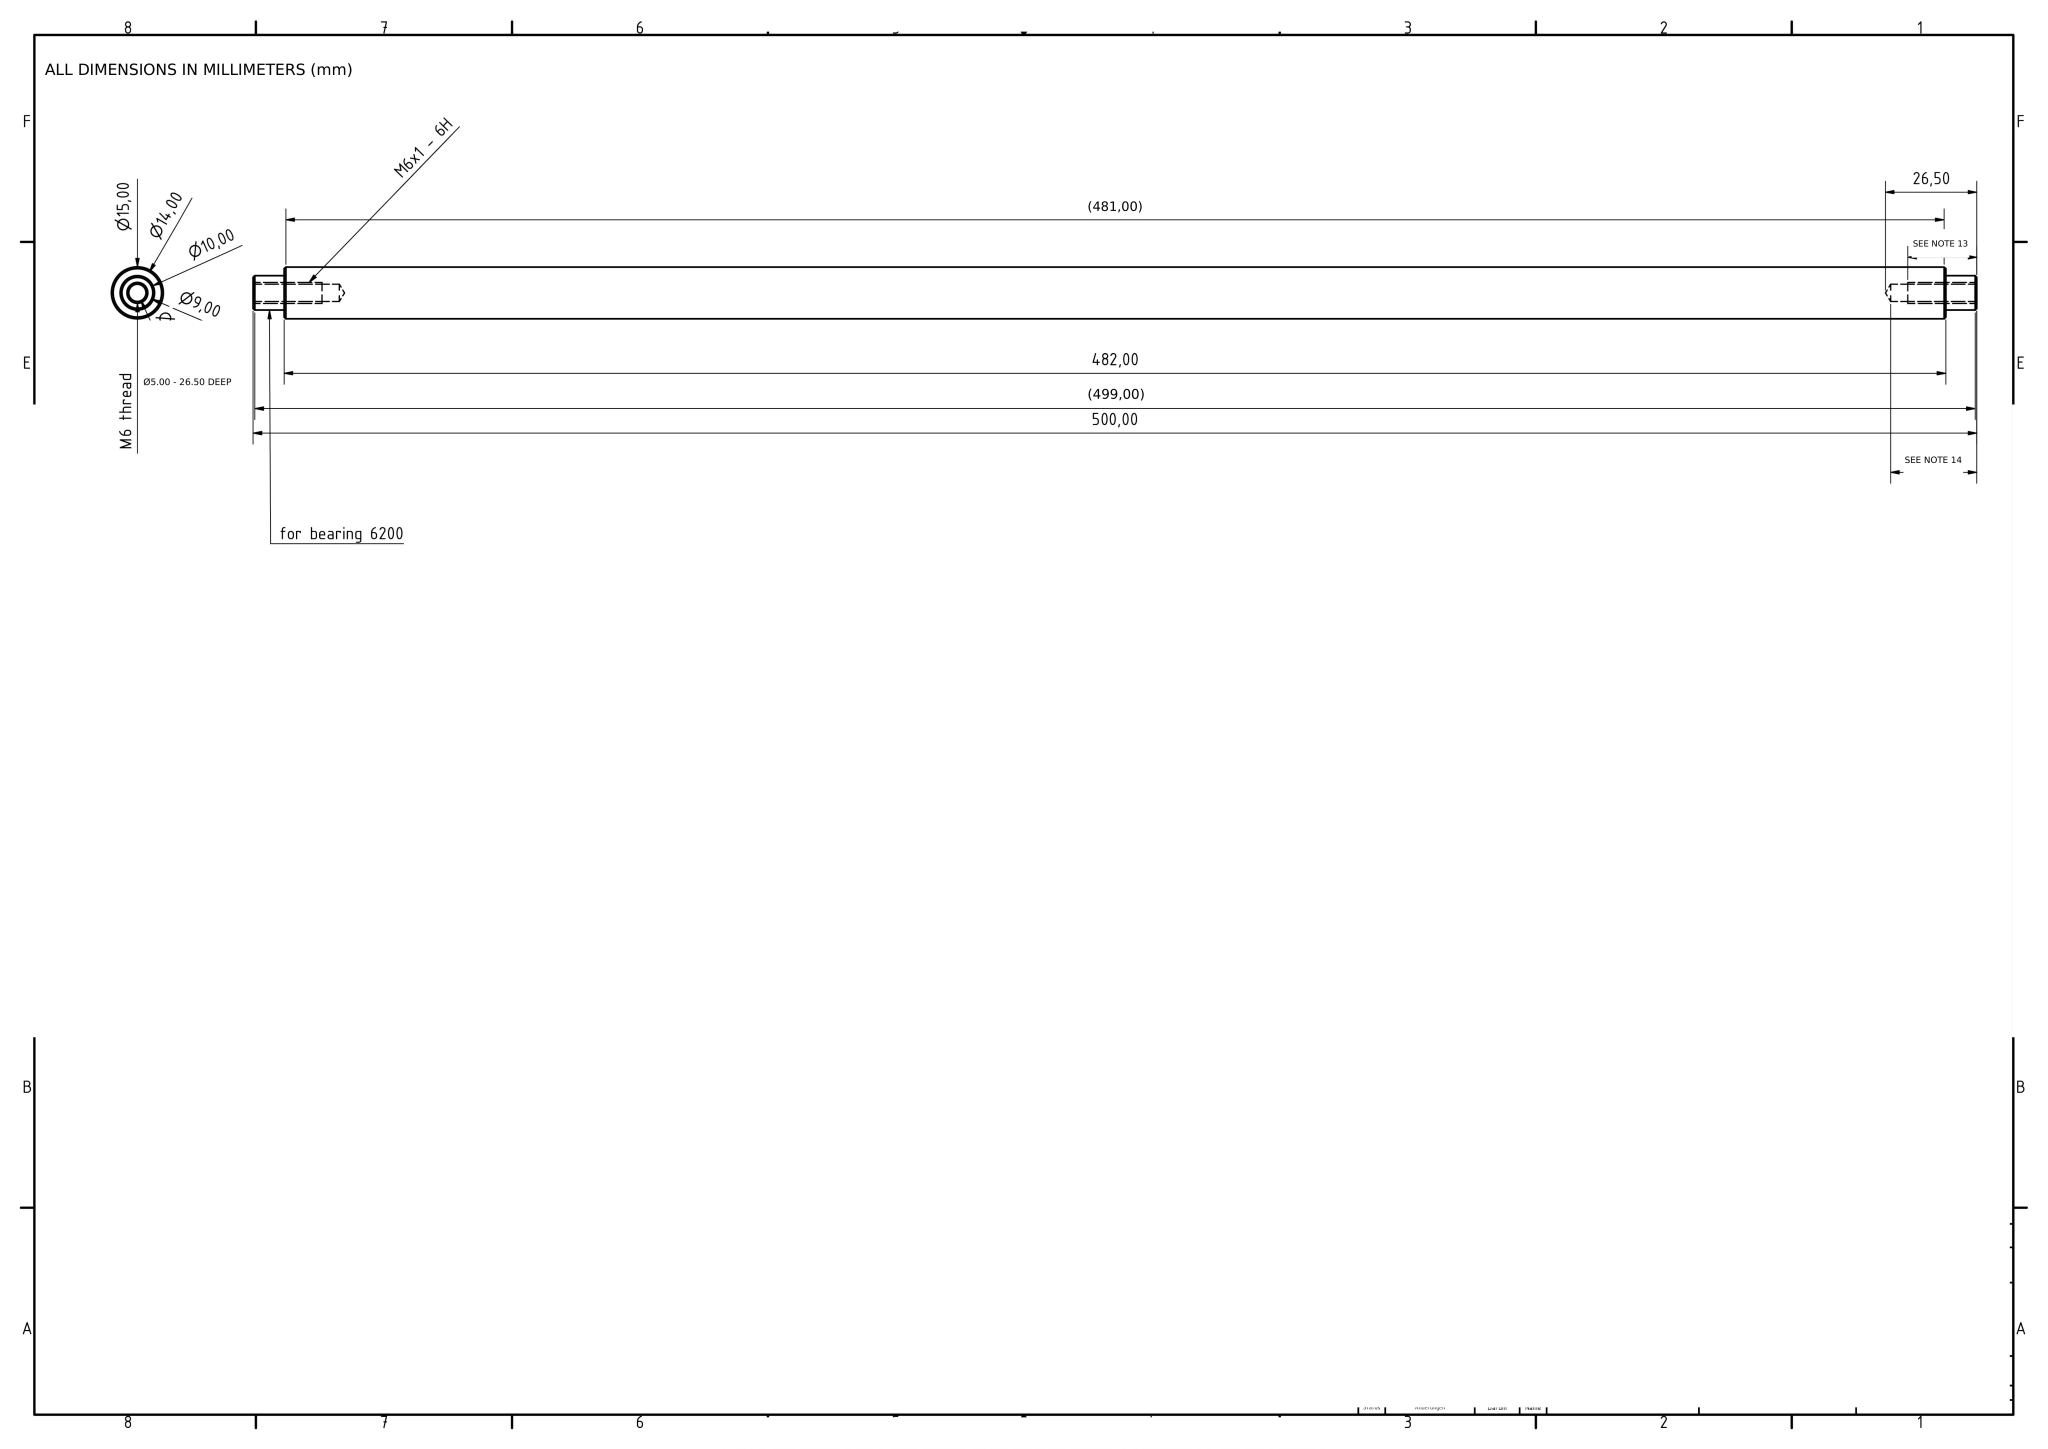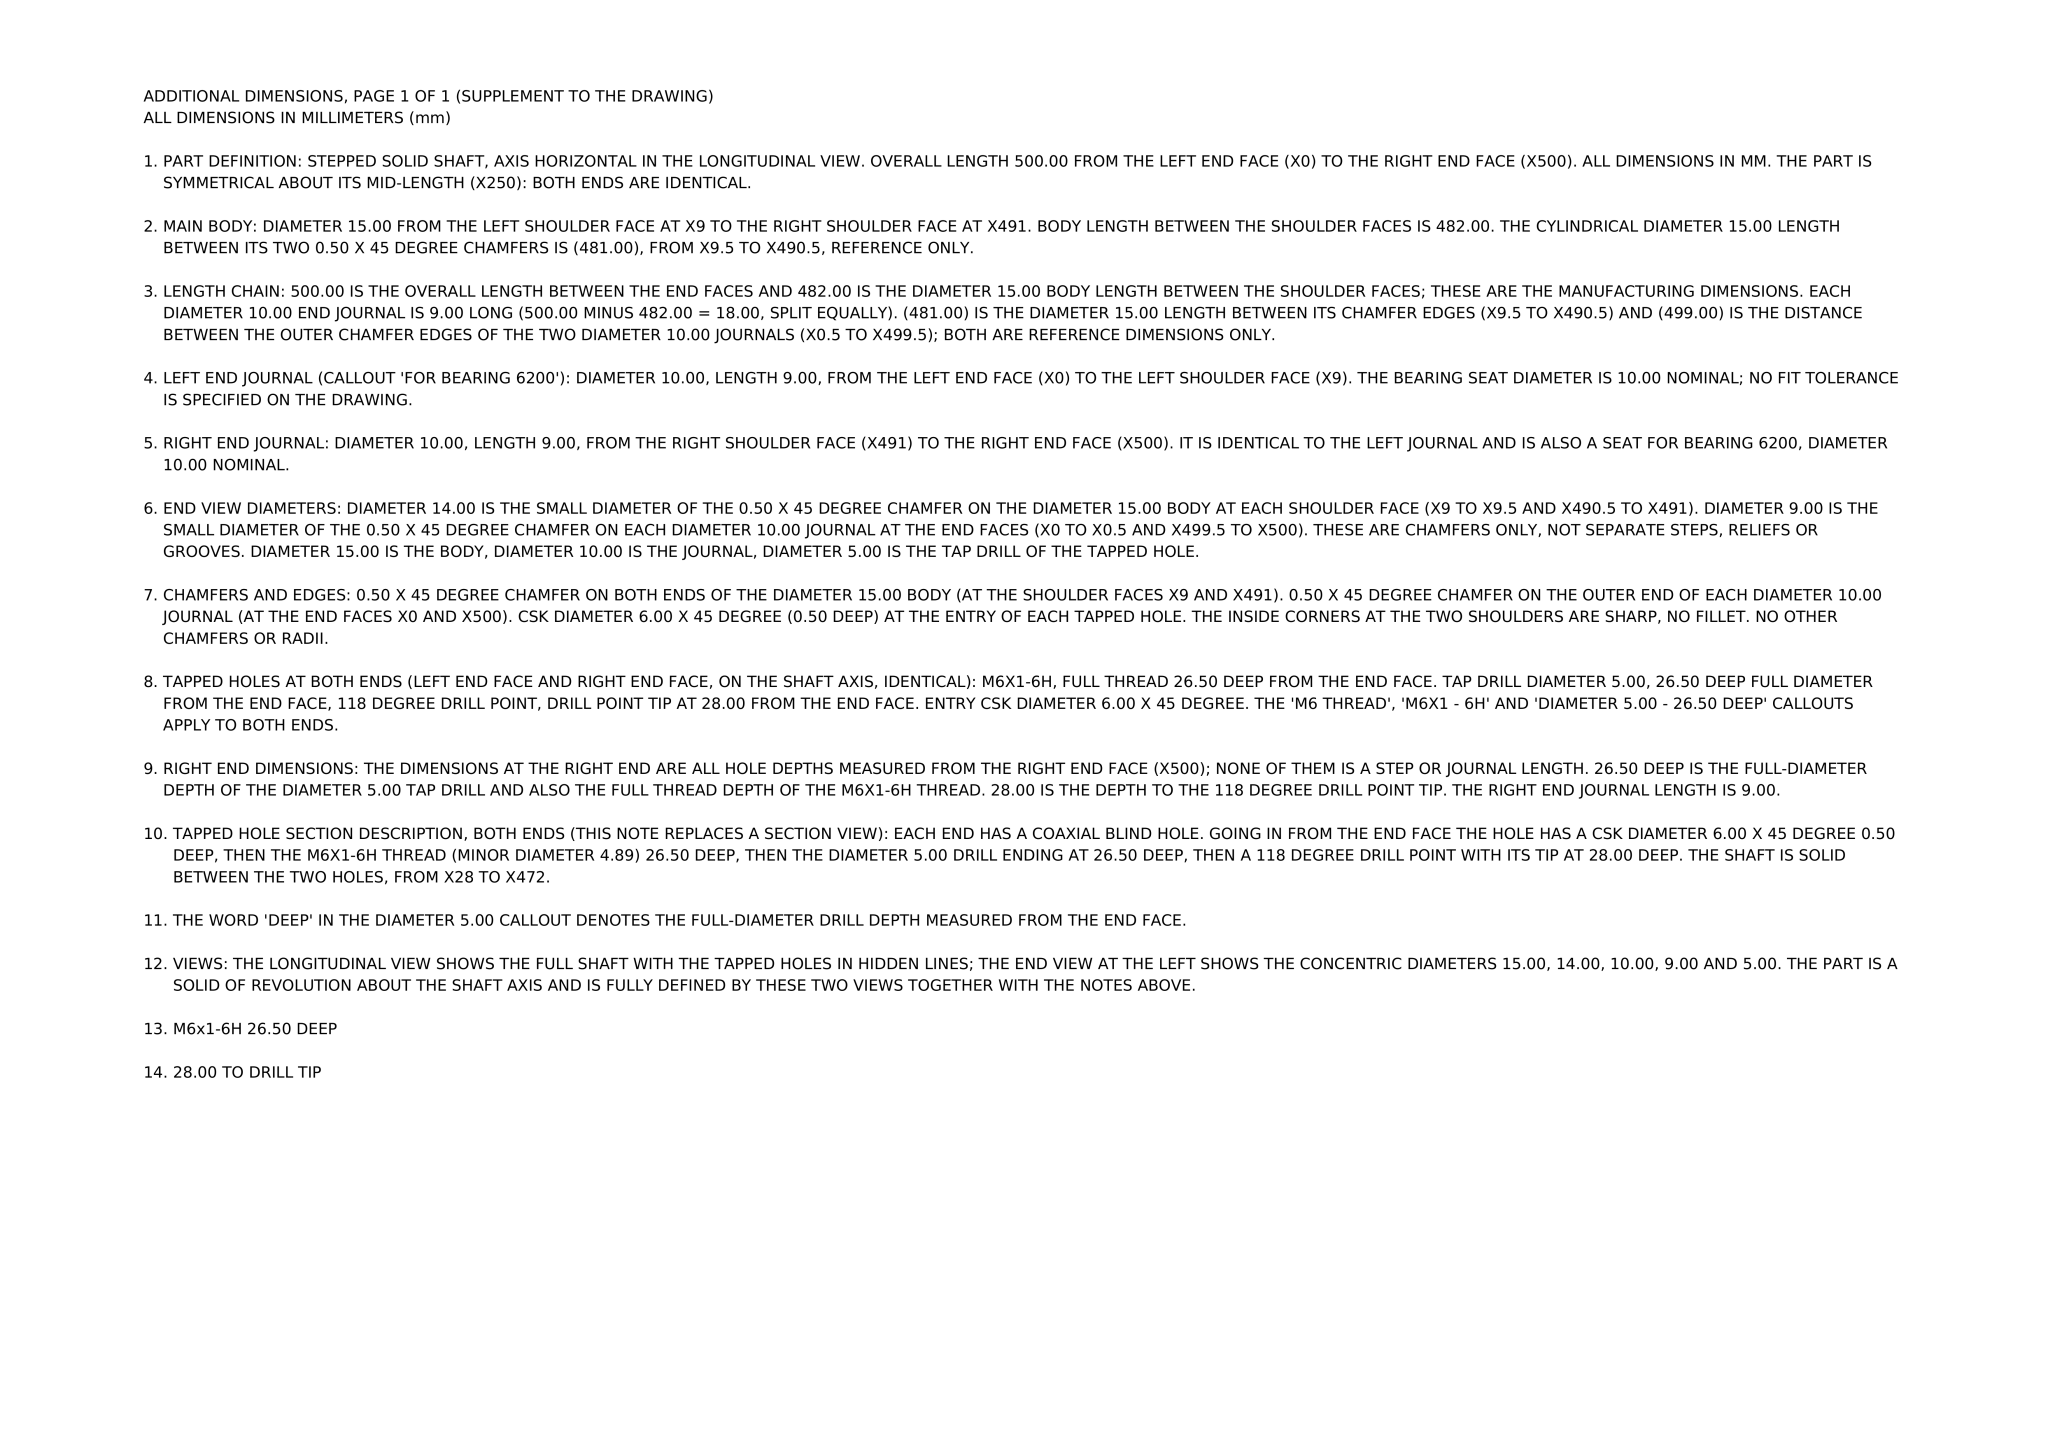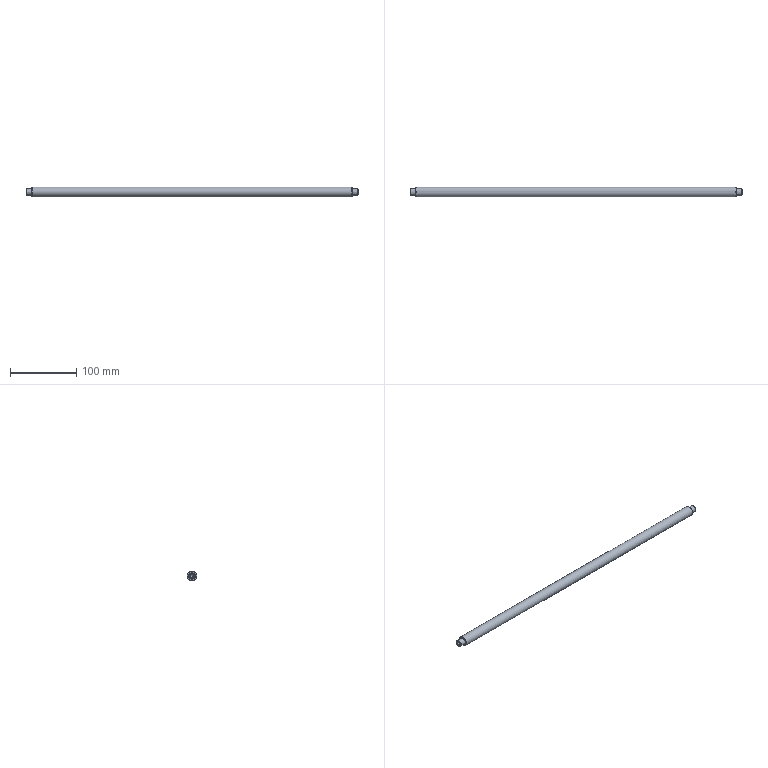Part | NX | mm | 1 solid | 17 faces | box 500 x 15 x 15 mm | volume 85565 mm3 | cone 8 | cylinder 5 | plane 4 | commonest cylinder face diameters 10 x2 5 x2 15 x1
STEP:
#1=(LENGTH_UNIT()NAMED_UNIT(*)SI_UNIT(.MILLI.,.METRE.));
#2=UNCERTAINTY_MEASURE_WITH_UNIT(LENGTH_MEASURE(0.000001),#1,'','');
#3=(NAMED_UNIT(*)PLANE_ANGLE_UNIT()SI_UNIT($,.RADIAN.));
#4=PLANE_ANGLE_MEASURE_WITH_UNIT(PLANE_ANGLE_MEASURE(0.01745),#3);
#5=DIMENSIONAL_EXPONENTS(0.,0.,0.,0.,0.,0.,0.);
#6=(CONVERSION_BASED_UNIT('',#4)NAMED_UNIT(#5)PLANE_ANGLE_UNIT());
#7=(NAMED_UNIT(*)SI_UNIT($,.STERADIAN.)SOLID_ANGLE_UNIT());
#8=(GEOMETRIC_REPRESENTATION_CONTEXT(3)GLOBAL_UNCERTAINTY_ASSIGNED_CONTEXT((#2))GLOBAL_UNIT_ASSIGNED_CONTEXT((#6,#7,#1))REPRESENTATION_CONTEXT('',''));
#9=COLOUR_RGB('',0.75,0.75,0.75);
#10=FILL_AREA_STYLE_COLOUR('',#9);
#11=FILL_AREA_STYLE('',(#10));
#12=SURFACE_STYLE_FILL_AREA(#11);
#13=SURFACE_SIDE_STYLE('',(#12));
#14=SURFACE_STYLE_USAGE(.BOTH.,#13);
#15=PRESENTATION_STYLE_ASSIGNMENT((#14));
#16=CARTESIAN_POINT('',(491.,7.,-0.));
#17=VERTEX_POINT('',#16);
#18=CARTESIAN_POINT('',(491.,0.,0.));
#19=DIRECTION('',(-1.,0.,0.));
#20=DIRECTION('',(0.,-1.,0.));
#21=AXIS2_PLACEMENT_3D('',#18,#19,#20);
#22=CIRCLE('',#21,7.);
#23=EDGE_CURVE('',#17,#17,#22,.T.);
#24=ORIENTED_EDGE('',*,*,#23,.T.);
#25=EDGE_LOOP('',(#24));
#26=FACE_OUTER_BOUND('',#25,.T.);
#27=CARTESIAN_POINT('',(490.5,7.5,0.));
#28=VERTEX_POINT('',#27);
#29=CARTESIAN_POINT('',(490.5,0.,0.));
#30=DIRECTION('',(1.,0.,0.));
#31=DIRECTION('',(0.,-1.,0.));
#32=AXIS2_PLACEMENT_3D('',#29,#30,#31);
#33=CIRCLE('',#32,7.5);
#34=EDGE_CURVE('',#28,#28,#33,.T.);
#35=ORIENTED_EDGE('',*,*,#34,.T.);
#36=EDGE_LOOP('',(#35));
#37=FACE_BOUND('',#36,.T.);
#38=CARTESIAN_POINT('',(490.75,0.,0.));
#39=DIRECTION('',(-1.,0.,0.));
#40=DIRECTION('',(0.,-1.,0.));
#41=AXIS2_PLACEMENT_3D('',#38,#39,#40);
#42=CONICAL_SURFACE('',#41,7.25,45.);
#43=ADVANCED_FACE('',(#26,#37),#42,.T.);
#44=CARTESIAN_POINT('',(9.5,7.5,-0.));
#45=VERTEX_POINT('',#44);
#46=CARTESIAN_POINT('',(9.5,0.,0.));
#47=DIRECTION('',(-1.,0.,0.));
#48=DIRECTION('',(0.,-1.,0.));
#49=AXIS2_PLACEMENT_3D('',#46,#47,#48);
#50=CIRCLE('',#49,7.5);
#51=EDGE_CURVE('',#45,#45,#50,.T.);
#52=ORIENTED_EDGE('',*,*,#51,.F.);
#53=EDGE_LOOP('',(#52));
#54=FACE_OUTER_BOUND('',#53,.T.);
#55=ORIENTED_EDGE('',*,*,#34,.F.);
#56=EDGE_LOOP('',(#55));
#57=FACE_BOUND('',#56,.T.);
#58=CARTESIAN_POINT('',(0.,0.,0.));
#59=DIRECTION('',(1.,0.,0.));
#60=DIRECTION('',(0.,-1.,0.));
#61=AXIS2_PLACEMENT_3D('',#58,#59,#60);
#62=CYLINDRICAL_SURFACE('',#61,7.5);
#63=ADVANCED_FACE('',(#54,#57),#62,.T.);
#64=ORIENTED_EDGE('',*,*,#23,.F.);
#65=EDGE_LOOP('',(#64));
#66=FACE_OUTER_BOUND('',#65,.T.);
#67=CARTESIAN_POINT('',(491.,0.,-5.));
#68=VERTEX_POINT('',#67);
#69=CARTESIAN_POINT('',(491.,0.,0.));
#70=DIRECTION('',(1.,0.,0.));
#71=DIRECTION('',(0.,0.,1.));
#72=AXIS2_PLACEMENT_3D('',#69,#70,#71);
#73=CIRCLE('',#72,5.);
#74=EDGE_CURVE('',#68,#68,#73,.T.);
#75=ORIENTED_EDGE('',*,*,#74,.F.);
#76=EDGE_LOOP('',(#75));
#77=FACE_BOUND('',#76,.T.);
#78=CARTESIAN_POINT('',(491.,0.,0.));
#79=DIRECTION('',(1.,0.,0.));
#80=DIRECTION('',(0.,0.,-1.));
#81=AXIS2_PLACEMENT_3D('',#78,#79,#80);
#82=PLANE('',#81);
#83=ADVANCED_FACE('',(#66,#77),#82,.T.);
#84=CARTESIAN_POINT('',(9.,7.,0.));
#85=VERTEX_POINT('',#84);
#86=CARTESIAN_POINT('',(9.,0.,0.));
#87=DIRECTION('',(1.,0.,0.));
#88=DIRECTION('',(0.,-1.,0.));
#89=AXIS2_PLACEMENT_3D('',#86,#87,#88);
#90=CIRCLE('',#89,7.);
#91=EDGE_CURVE('',#85,#85,#90,.T.);
#92=ORIENTED_EDGE('',*,*,#91,.T.);
#93=EDGE_LOOP('',(#92));
#94=FACE_OUTER_BOUND('',#93,.T.);
#95=ORIENTED_EDGE('',*,*,#51,.T.);
#96=EDGE_LOOP('',(#95));
#97=FACE_BOUND('',#96,.T.);
#98=CARTESIAN_POINT('',(9.25,0.,0.));
#99=DIRECTION('',(1.,0.,0.));
#100=DIRECTION('',(0.,-1.,0.));
#101=AXIS2_PLACEMENT_3D('',#98,#99,#100);
#102=CONICAL_SURFACE('',#101,7.25,45.);
#103=ADVANCED_FACE('',(#94,#97),#102,.T.);
#104=ORIENTED_EDGE('',*,*,#91,.F.);
#105=EDGE_LOOP('',(#104));
#106=FACE_OUTER_BOUND('',#105,.T.);
#107=CARTESIAN_POINT('',(9.,0.,5.));
#108=VERTEX_POINT('',#107);
#109=CARTESIAN_POINT('',(9.,0.,0.));
#110=DIRECTION('',(-1.,0.,0.));
#111=DIRECTION('',(0.,0.,-1.));
#112=AXIS2_PLACEMENT_3D('',#109,#110,#111);
#113=CIRCLE('',#112,5.);
#114=EDGE_CURVE('',#108,#108,#113,.T.);
#115=ORIENTED_EDGE('',*,*,#114,.F.);
#116=EDGE_LOOP('',(#115));
#117=FACE_BOUND('',#116,.T.);
#118=CARTESIAN_POINT('',(9.,0.,-0.));
#119=DIRECTION('',(1.,0.,0.));
#120=DIRECTION('',(0.,0.,-1.));
#121=AXIS2_PLACEMENT_3D('',#118,#119,#120);
#122=PLANE('',#121);
#123=ADVANCED_FACE('',(#106,#117),#122,.F.);
#124=CARTESIAN_POINT('',(499.5,0.,-5.));
#125=VERTEX_POINT('',#124);
#126=CARTESIAN_POINT('',(499.5,0.,0.));
#127=DIRECTION('',(1.,0.,0.));
#128=DIRECTION('',(0.,0.,1.));
#129=AXIS2_PLACEMENT_3D('',#126,#127,#128);
#130=CIRCLE('',#129,5.);
#131=EDGE_CURVE('',#125,#125,#130,.T.);
#132=ORIENTED_EDGE('',*,*,#131,.T.);
#133=EDGE_LOOP('',(#132));
#134=FACE_OUTER_BOUND('',#133,.T.);
#135=CARTESIAN_POINT('',(500.,-0.,-4.5));
#136=VERTEX_POINT('',#135);
#137=CARTESIAN_POINT('',(500.,0.,0.));
#138=DIRECTION('',(-1.,0.,0.));
#139=DIRECTION('',(0.,0.,1.));
#140=AXIS2_PLACEMENT_3D('',#137,#138,#139);
#141=CIRCLE('',#140,4.5);
#142=EDGE_CURVE('',#136,#136,#141,.T.);
#143=ORIENTED_EDGE('',*,*,#142,.T.);
#144=EDGE_LOOP('',(#143));
#145=FACE_BOUND('',#144,.T.);
#146=CARTESIAN_POINT('',(499.75,0.,0.));
#147=DIRECTION('',(-1.,0.,0.));
#148=DIRECTION('',(0.,0.,1.));
#149=AXIS2_PLACEMENT_3D('',#146,#147,#148);
#150=CONICAL_SURFACE('',#149,4.75,45.);
#151=ADVANCED_FACE('',(#134,#145),#150,.T.);
#152=ORIENTED_EDGE('',*,*,#142,.F.);
#153=EDGE_LOOP('',(#152));
#154=FACE_OUTER_BOUND('',#153,.T.);
#155=CARTESIAN_POINT('',(500.,0.,-3.));
#156=VERTEX_POINT('',#155);
#157=CARTESIAN_POINT('',(500.,0.,0.));
#158=DIRECTION('',(1.,0.,0.));
#159=DIRECTION('',(0.,0.,1.));
#160=AXIS2_PLACEMENT_3D('',#157,#158,#159);
#161=CIRCLE('',#160,3.);
#162=EDGE_CURVE('',#156,#156,#161,.T.);
#163=ORIENTED_EDGE('',*,*,#162,.F.);
#164=EDGE_LOOP('',(#163));
#165=FACE_BOUND('',#164,.T.);
#166=CARTESIAN_POINT('',(500.,-0.,0.));
#167=DIRECTION('',(1.,0.,0.));
#168=DIRECTION('',(0.,0.,-1.));
#169=AXIS2_PLACEMENT_3D('',#166,#167,#168);
#170=PLANE('',#169);
#171=ADVANCED_FACE('',(#154,#165),#170,.T.);
#172=ORIENTED_EDGE('',*,*,#74,.T.);
#173=EDGE_LOOP('',(#172));
#174=FACE_OUTER_BOUND('',#173,.T.);
#175=ORIENTED_EDGE('',*,*,#131,.F.);
#176=EDGE_LOOP('',(#175));
#177=FACE_BOUND('',#176,.T.);
#178=CARTESIAN_POINT('',(500.,0.,0.));
#179=DIRECTION('',(-1.,0.,0.));
#180=DIRECTION('',(0.,0.,1.));
#181=AXIS2_PLACEMENT_3D('',#178,#179,#180);
#182=CYLINDRICAL_SURFACE('',#181,5.);
#183=ADVANCED_FACE('',(#174,#177),#182,.T.);
#184=CARTESIAN_POINT('',(499.5,-0.,-2.5));
#185=VERTEX_POINT('',#184);
#186=CARTESIAN_POINT('',(499.5,0.,0.));
#187=DIRECTION('',(-1.,0.,0.));
#188=DIRECTION('',(0.,0.,1.));
#189=AXIS2_PLACEMENT_3D('',#186,#187,#188);
#190=CIRCLE('',#189,2.5);
#191=EDGE_CURVE('',#185,#185,#190,.T.);
#192=ORIENTED_EDGE('',*,*,#191,.T.);
#193=EDGE_LOOP('',(#192));
#194=FACE_OUTER_BOUND('',#193,.T.);
#195=ORIENTED_EDGE('',*,*,#162,.T.);
#196=EDGE_LOOP('',(#195));
#197=FACE_BOUND('',#196,.T.);
#198=CARTESIAN_POINT('',(499.75,0.,0.));
#199=DIRECTION('',(1.,0.,0.));
#200=DIRECTION('',(0.,0.,1.));
#201=AXIS2_PLACEMENT_3D('',#198,#199,#200);
#202=CONICAL_SURFACE('',#201,2.75,45.);
#203=ADVANCED_FACE('',(#194,#197),#202,.F.);
#204=CARTESIAN_POINT('',(475.,0.,-2.5));
#205=VERTEX_POINT('',#204);
#206=CARTESIAN_POINT('',(475.,0.,0.));
#207=DIRECTION('',(1.,0.,0.));
#208=DIRECTION('',(0.,0.,-1.));
#209=AXIS2_PLACEMENT_3D('',#206,#207,#208);
#210=CIRCLE('',#209,2.5);
#211=EDGE_CURVE('',#205,#205,#210,.T.);
#212=ORIENTED_EDGE('',*,*,#211,.F.);
#213=EDGE_LOOP('',(#212));
#214=FACE_OUTER_BOUND('',#213,.T.);
#215=ORIENTED_EDGE('',*,*,#191,.F.);
#216=EDGE_LOOP('',(#215));
#217=FACE_BOUND('',#216,.T.);
#218=CARTESIAN_POINT('',(487.5,0.,0.));
#219=DIRECTION('',(1.,0.,0.));
#220=DIRECTION('',(0.,0.,-1.));
#221=AXIS2_PLACEMENT_3D('',#218,#219,#220);
#222=CYLINDRICAL_SURFACE('',#221,2.5);
#223=ADVANCED_FACE('',(#214,#217),#222,.F.);
#224=CARTESIAN_POINT('',(0.5,-0.,2.5));
#225=VERTEX_POINT('',#224);
#226=CARTESIAN_POINT('',(0.5,0.,0.));
#227=DIRECTION('',(1.,0.,0.));
#228=DIRECTION('',(0.,0.,-1.));
#229=AXIS2_PLACEMENT_3D('',#226,#227,#228);
#230=CIRCLE('',#229,2.5);
#231=EDGE_CURVE('',#225,#225,#230,.T.);
#232=ORIENTED_EDGE('',*,*,#231,.T.);
#233=EDGE_LOOP('',(#232));
#234=FACE_OUTER_BOUND('',#233,.T.);
#235=CARTESIAN_POINT('',(0.,0.,3.));
#236=VERTEX_POINT('',#235);
#237=CARTESIAN_POINT('',(0.,0.,0.));
#238=DIRECTION('',(-1.,0.,0.));
#239=DIRECTION('',(0.,0.,-1.));
#240=AXIS2_PLACEMENT_3D('',#237,#238,#239);
#241=CIRCLE('',#240,3.);
#242=EDGE_CURVE('',#236,#236,#241,.T.);
#243=ORIENTED_EDGE('',*,*,#242,.T.);
#244=EDGE_LOOP('',(#243));
#245=FACE_BOUND('',#244,.T.);
#246=CARTESIAN_POINT('',(0.25,0.,0.));
#247=DIRECTION('',(-1.,0.,0.));
#248=DIRECTION('',(0.,0.,-1.));
#249=AXIS2_PLACEMENT_3D('',#246,#247,#248);
#250=CONICAL_SURFACE('',#249,2.75,45.);
#251=ADVANCED_FACE('',(#234,#245),#250,.F.);
#252=CARTESIAN_POINT('',(0.,-0.,4.5));
#253=VERTEX_POINT('',#252);
#254=CARTESIAN_POINT('',(0.,0.,0.));
#255=DIRECTION('',(1.,0.,0.));
#256=DIRECTION('',(0.,0.,-1.));
#257=AXIS2_PLACEMENT_3D('',#254,#255,#256);
#258=CIRCLE('',#257,4.5);
#259=EDGE_CURVE('',#253,#253,#258,.T.);
#260=ORIENTED_EDGE('',*,*,#259,.F.);
#261=EDGE_LOOP('',(#260));
#262=FACE_OUTER_BOUND('',#261,.T.);
#263=ORIENTED_EDGE('',*,*,#242,.F.);
#264=EDGE_LOOP('',(#263));
#265=FACE_BOUND('',#264,.T.);
#266=CARTESIAN_POINT('',(0.,-0.,0.));
#267=DIRECTION('',(1.,0.,0.));
#268=DIRECTION('',(0.,0.,-1.));
#269=AXIS2_PLACEMENT_3D('',#266,#267,#268);
#270=PLANE('',#269);
#271=ADVANCED_FACE('',(#262,#265),#270,.F.);
#272=CARTESIAN_POINT('',(25.,0.,2.5));
#273=VERTEX_POINT('',#272);
#274=CARTESIAN_POINT('',(25.,0.,0.));
#275=DIRECTION('',(-1.,0.,0.));
#276=DIRECTION('',(0.,0.,1.));
#277=AXIS2_PLACEMENT_3D('',#274,#275,#276);
#278=CIRCLE('',#277,2.5);
#279=EDGE_CURVE('',#273,#273,#278,.T.);
#280=ORIENTED_EDGE('',*,*,#279,.F.);
#281=EDGE_LOOP('',(#280));
#282=FACE_OUTER_BOUND('',#281,.T.);
#283=ORIENTED_EDGE('',*,*,#231,.F.);
#284=EDGE_LOOP('',(#283));
#285=FACE_BOUND('',#284,.T.);
#286=CARTESIAN_POINT('',(12.5,0.,0.));
#287=DIRECTION('',(-1.,0.,0.));
#288=DIRECTION('',(0.,0.,1.));
#289=AXIS2_PLACEMENT_3D('',#286,#287,#288);
#290=CYLINDRICAL_SURFACE('',#289,2.5);
#291=ADVANCED_FACE('',(#282,#285),#290,.F.);
#292=CARTESIAN_POINT('',(0.5,0.,5.));
#293=VERTEX_POINT('',#292);
#294=CARTESIAN_POINT('',(0.5,0.,0.));
#295=DIRECTION('',(-1.,0.,0.));
#296=DIRECTION('',(0.,0.,-1.));
#297=AXIS2_PLACEMENT_3D('',#294,#295,#296);
#298=CIRCLE('',#297,5.);
#299=EDGE_CURVE('',#293,#293,#298,.T.);
#300=ORIENTED_EDGE('',*,*,#299,.T.);
#301=EDGE_LOOP('',(#300));
#302=FACE_OUTER_BOUND('',#301,.T.);
#303=ORIENTED_EDGE('',*,*,#259,.T.);
#304=EDGE_LOOP('',(#303));
#305=FACE_BOUND('',#304,.T.);
#306=CARTESIAN_POINT('',(0.25,0.,0.));
#307=DIRECTION('',(1.,0.,0.));
#308=DIRECTION('',(0.,0.,-1.));
#309=AXIS2_PLACEMENT_3D('',#306,#307,#308);
#310=CONICAL_SURFACE('',#309,4.75,45.);
#311=ADVANCED_FACE('',(#302,#305),#310,.T.);
#312=ORIENTED_EDGE('',*,*,#114,.T.);
#313=EDGE_LOOP('',(#312));
#314=FACE_OUTER_BOUND('',#313,.T.);
#315=ORIENTED_EDGE('',*,*,#299,.F.);
#316=EDGE_LOOP('',(#315));
#317=FACE_BOUND('',#316,.T.);
#318=CARTESIAN_POINT('',(0.,0.,0.));
#319=DIRECTION('',(1.,0.,0.));
#320=DIRECTION('',(0.,0.,-1.));
#321=AXIS2_PLACEMENT_3D('',#318,#319,#320);
#322=CYLINDRICAL_SURFACE('',#321,5.);
#323=ADVANCED_FACE('',(#314,#317),#322,.T.);
#324=ORIENTED_EDGE('',*,*,#211,.T.);
#325=EDGE_LOOP('',(#324));
#326=FACE_OUTER_BOUND('',#325,.T.);
#327=CARTESIAN_POINT('',(474.249,0.,0.));
#328=DIRECTION('',(1.,0.,0.));
#329=DIRECTION('',(0.,0.,-1.));
#330=AXIS2_PLACEMENT_3D('',#327,#328,#329);
#331=CONICAL_SURFACE('',#330,1.25,59.);
#332=ADVANCED_FACE('',(#326),#331,.F.);
#333=ORIENTED_EDGE('',*,*,#279,.T.);
#334=EDGE_LOOP('',(#333));
#335=FACE_OUTER_BOUND('',#334,.T.);
#336=CARTESIAN_POINT('',(25.751,0.,0.));
#337=DIRECTION('',(-1.,0.,0.));
#338=DIRECTION('',(0.,0.,1.));
#339=AXIS2_PLACEMENT_3D('',#336,#337,#338);
#340=CONICAL_SURFACE('',#339,1.25,59.);
#341=ADVANCED_FACE('',(#335),#340,.F.);
#342=CLOSED_SHELL('',(#43,#63,#83,#103,#123,#151,#171,#183,#203,#223,#251,#271,#291,#311,#323,#332,#341));
#343=MANIFOLD_SOLID_BREP('',#342);
#344=STYLED_ITEM('',(#15),#343);
#345=(LENGTH_UNIT()NAMED_UNIT(*)SI_UNIT(.MILLI.,.METRE.));
#346=UNCERTAINTY_MEASURE_WITH_UNIT(LENGTH_MEASURE(0.01),#345,'','');
#347=(NAMED_UNIT(*)PLANE_ANGLE_UNIT()SI_UNIT($,.RADIAN.));
#348=PLANE_ANGLE_MEASURE_WITH_UNIT(PLANE_ANGLE_MEASURE(0.01745),#347);
#349=DIMENSIONAL_EXPONENTS(0.,0.,0.,0.,0.,0.,0.);
#350=(CONVERSION_BASED_UNIT('',#348)NAMED_UNIT(#349)PLANE_ANGLE_UNIT());
#351=(NAMED_UNIT(*)SI_UNIT($,.STERADIAN.)SOLID_ANGLE_UNIT());
#352=(GEOMETRIC_REPRESENTATION_CONTEXT(3)GLOBAL_UNCERTAINTY_ASSIGNED_CONTEXT((#346))GLOBAL_UNIT_ASSIGNED_CONTEXT((#350,#351,#345))REPRESENTATION_CONTEXT('',''));
#353=MECHANICAL_DESIGN_GEOMETRIC_PRESENTATION_REPRESENTATION('',(#344),#352);
#354=ADVANCED_BREP_SHAPE_REPRESENTATION('',(#343),#352);
#355=CARTESIAN_POINT('',(0.,0.,0.));
#356=DIRECTION('',(0.,0.,1.));
#357=DIRECTION('',(1.,0.,0.));
#358=AXIS2_PLACEMENT_3D('',#355,#356,#357);
#359=SHAPE_REPRESENTATION('',(#358),#352);
#360=SHAPE_REPRESENTATION_RELATIONSHIP('','',#354,#359);